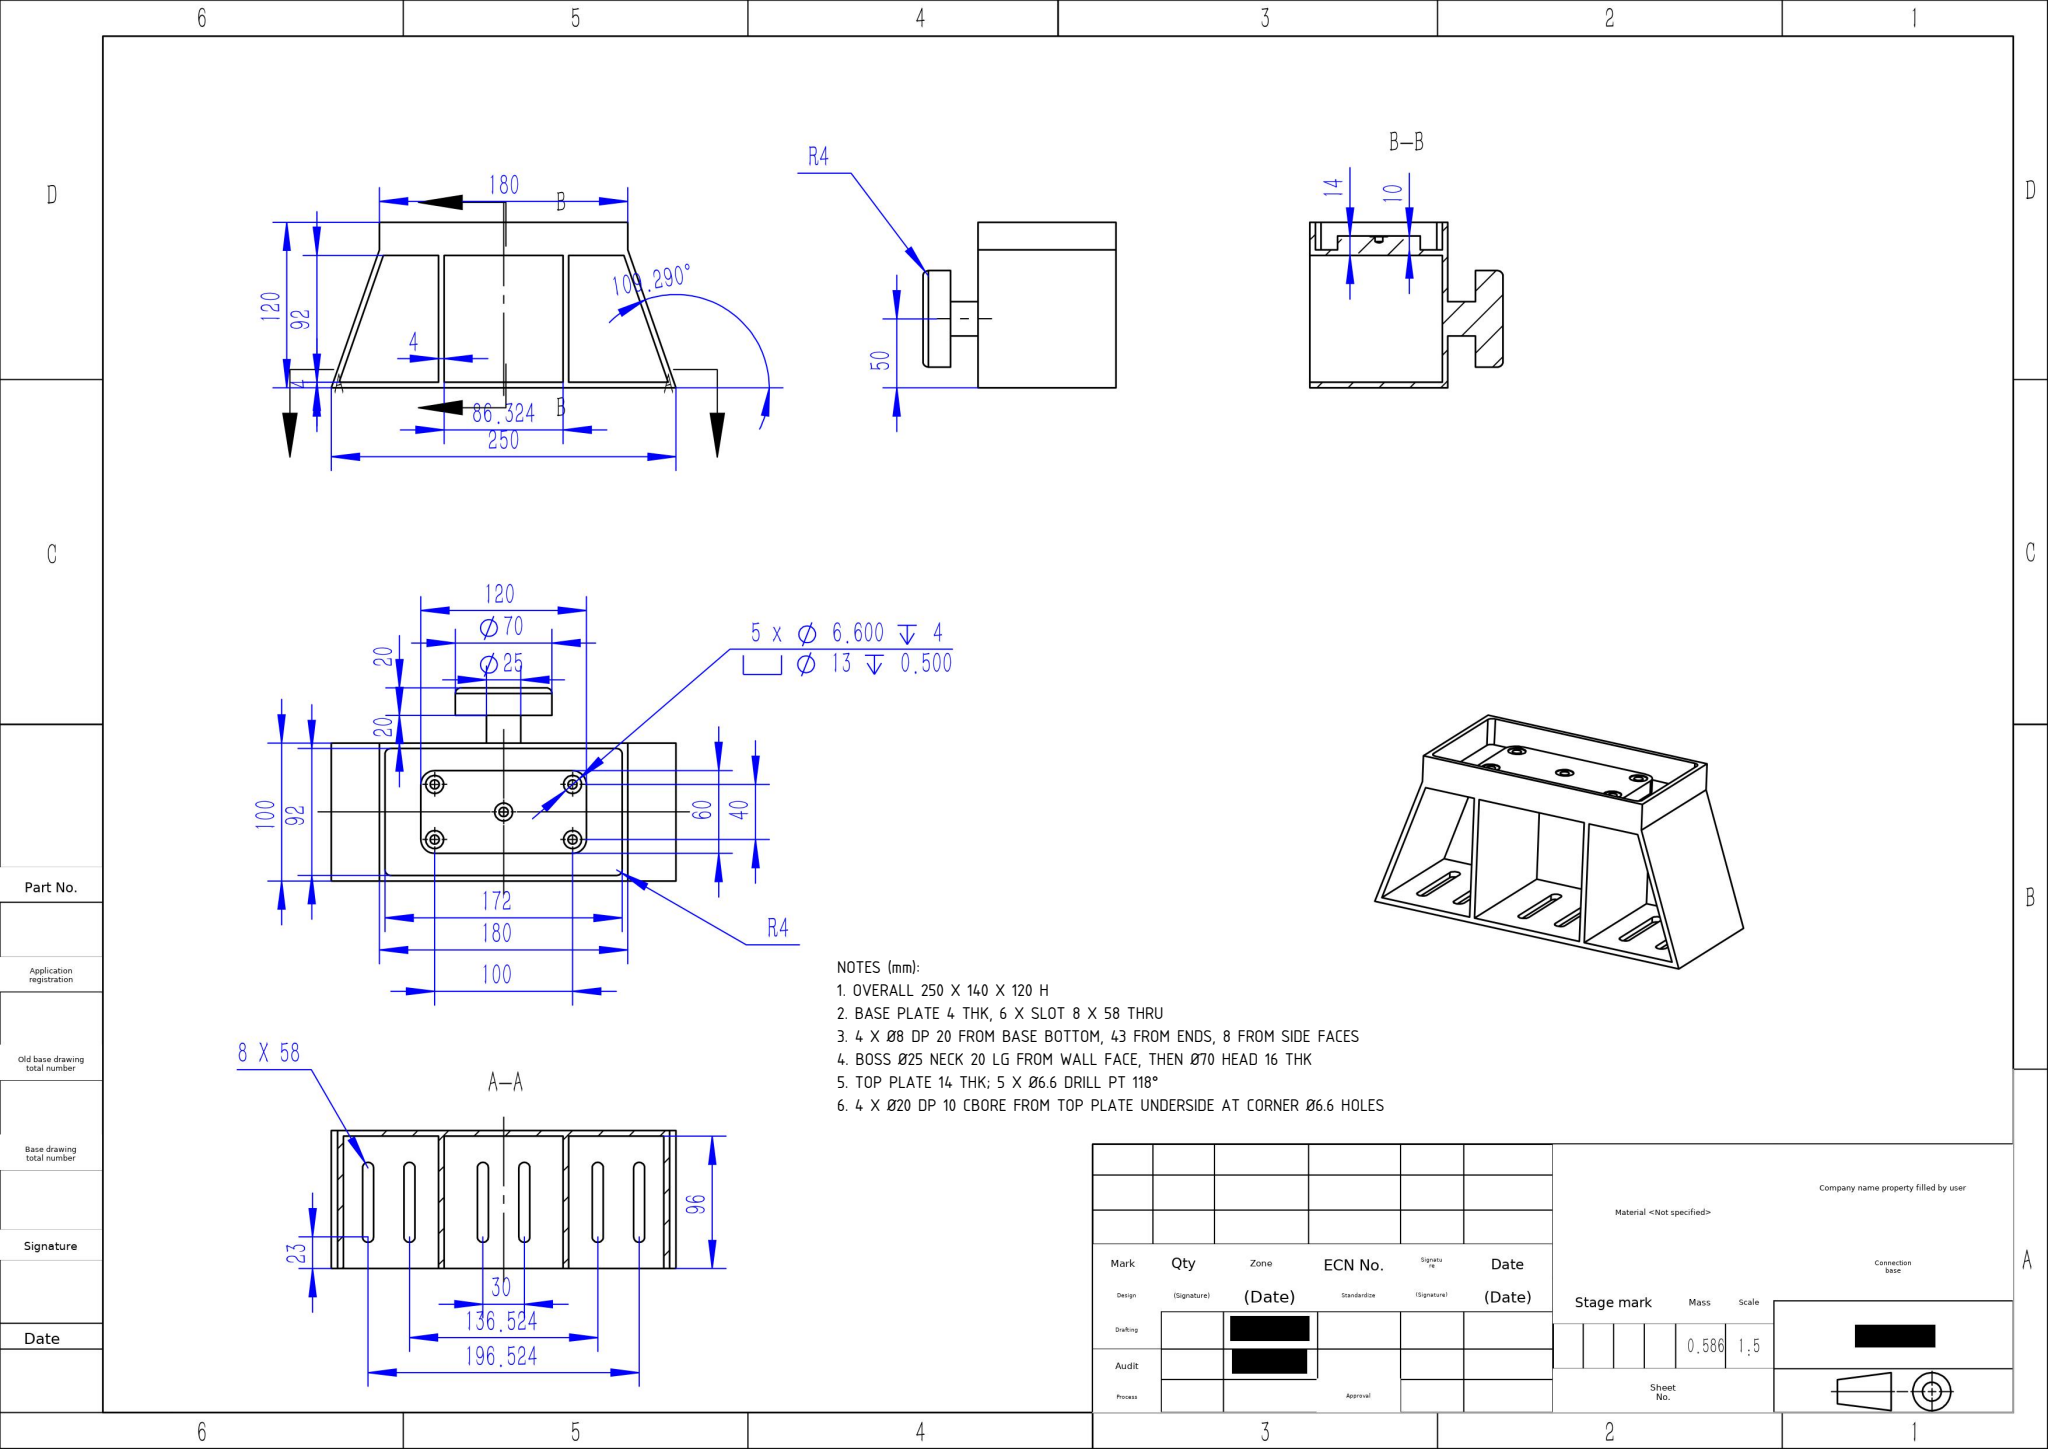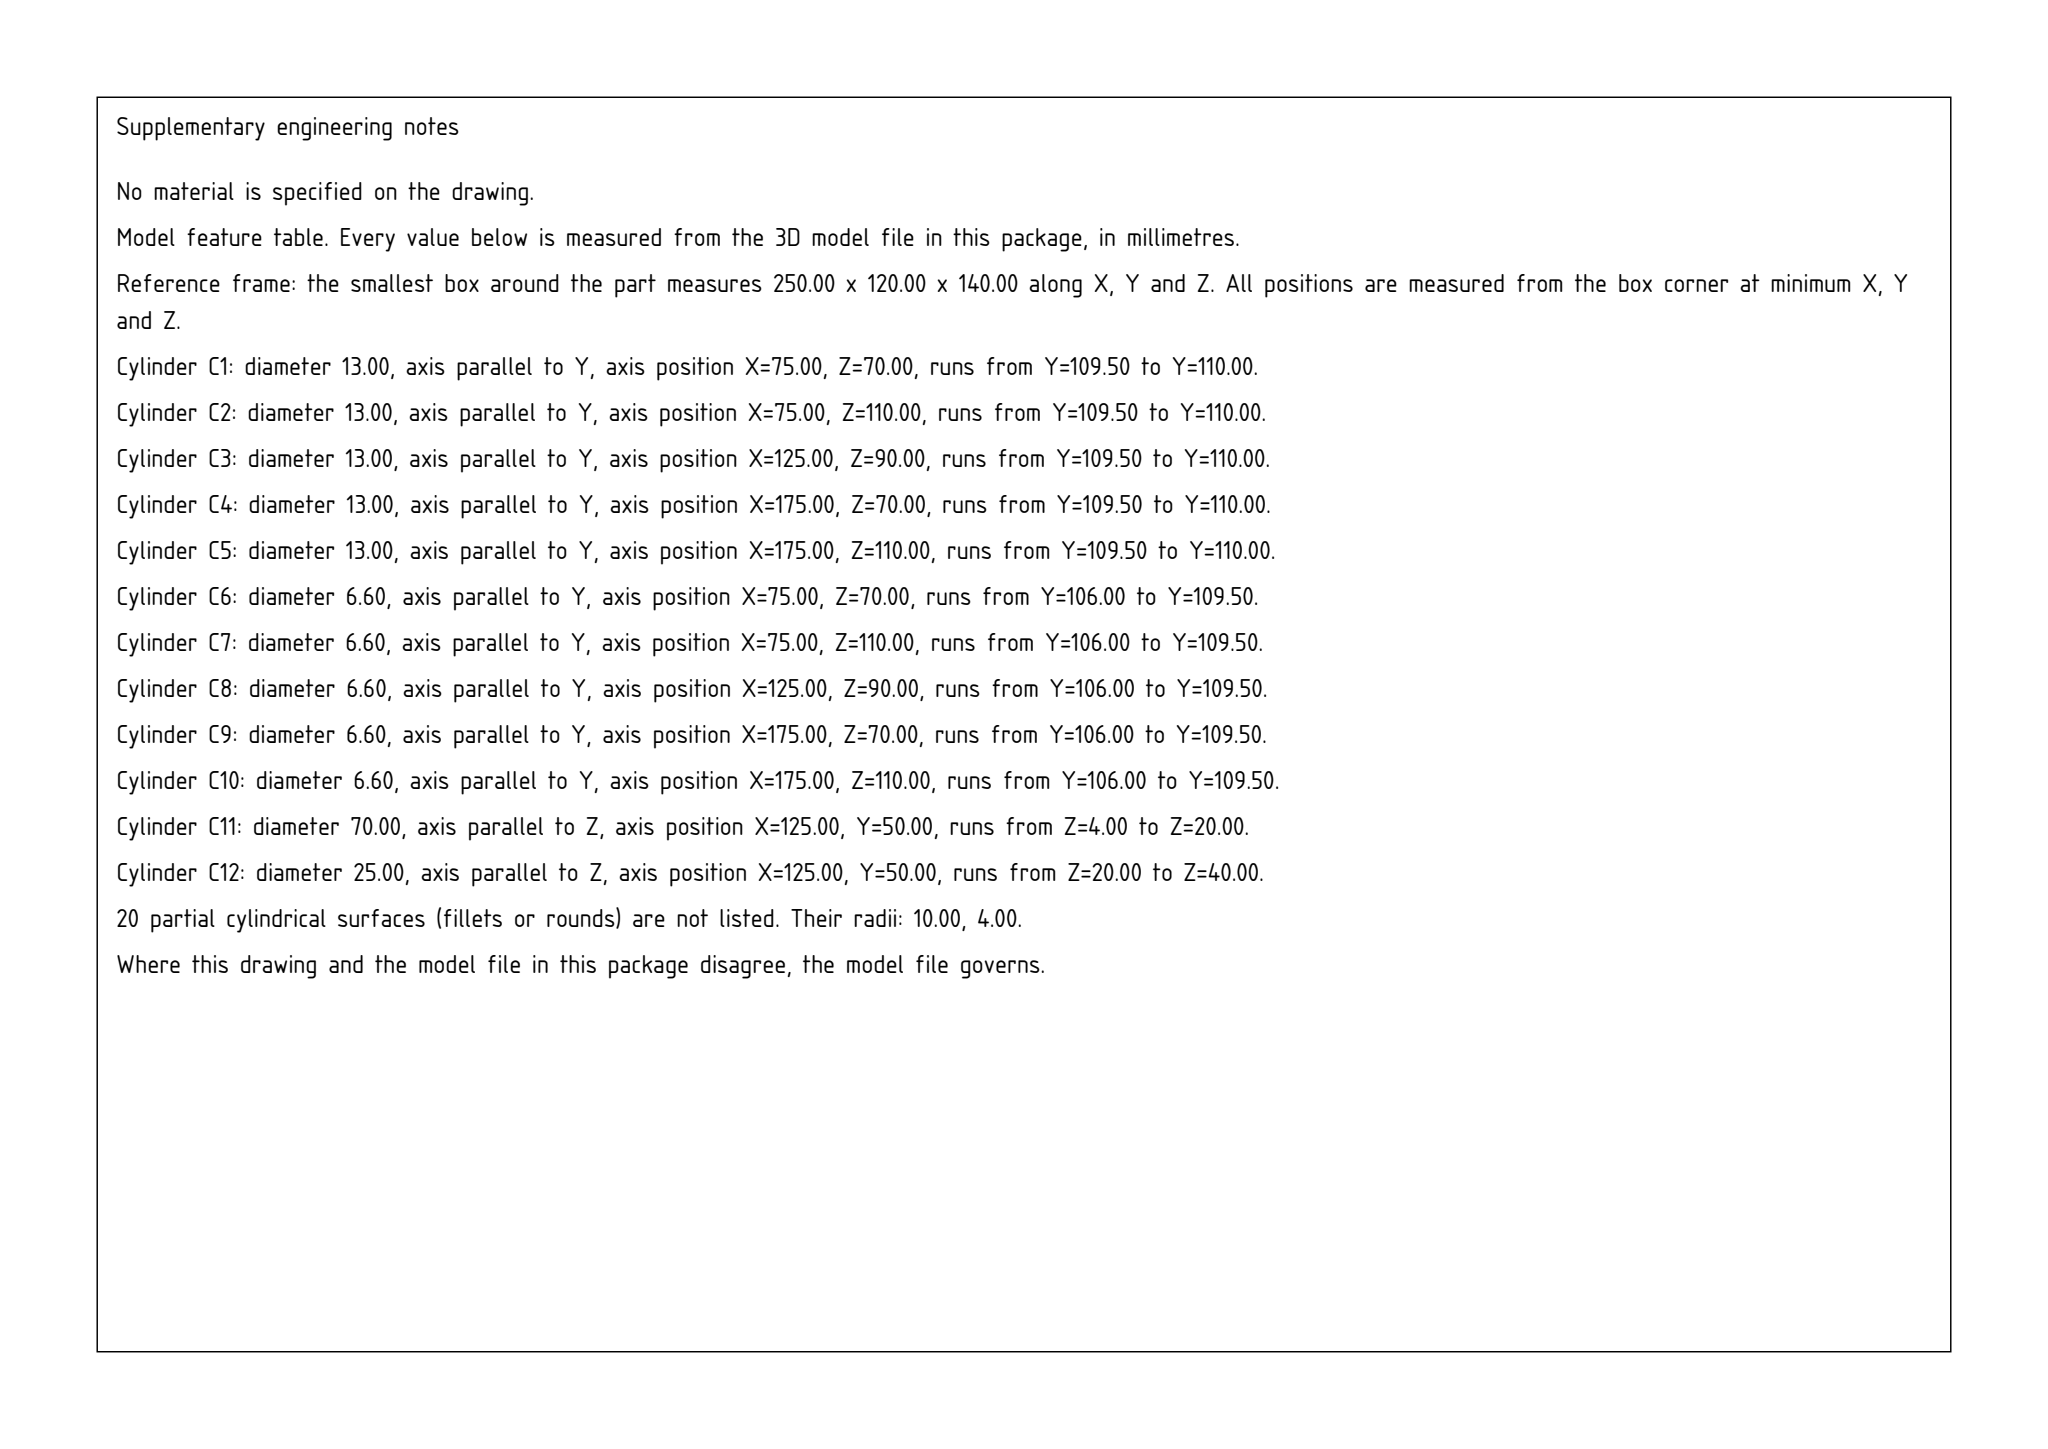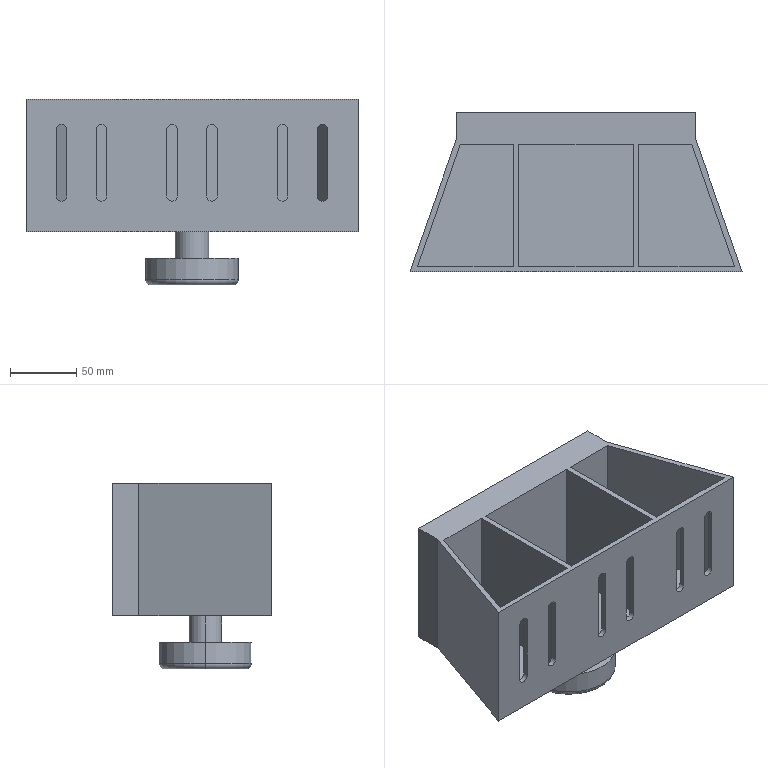Part | SolidWorks | mm | 1 solid | 108 faces | box 250 x 120 x 140 mm | volume 585772 mm3 | plane 52 | cylinder 44 | cone 10 | torus 2 | commonest cylinder face diameters 8 x16 13 x10 6.6 x10 20 x4 70 x2 25 x2
Drawing notes:
OVERALL 250 X 140 X 120 H | from the solid: bbox_xyz 250 x 120 x 140
BASE PLATE 4 THK, 6 X SLOT 8 X 58 THRU | from the solid: Ø8 y-axis cyls L=4 at z=67 & 117 (58 over ends), x=26.74/56.74, 110/140, 193.26/223.26; y planes 0 & 4
4 X Ø8 DP 20 FROM BASE BOTTOM, 43 FROM ENDS, 8 FROM SIDE FACES | from the solid: Ø8 y-axis cyls L=20 at x=43 & 207, z=48 & 132 (outer faces z=40/140), y 0-20
BOSS Ø25 NECK 20 LG FROM WALL FACE, THEN Ø70 HEAD 16 THK | from the solid: Ø25 z-axis cyl L=20 and Ø70 z-axis cyl L=16 at x=125, y=50; wall face z=40, step z=20
TOP PLATE 14 THK; 5 X Ø6.6 DRILL PT 118° | from the solid: y planes 96 (underside) & 110 (top) = 14 thk; cone 118° on Ø6.6 holes
4 X Ø20 DP 10 CBORE FROM TOP PLATE UNDERSIDE AT CORNER Ø6.6 HOLES | from the solid: Ø20 y-axis cyls L=10 at (x,z)=(75,70),(75,110),(175,70),(175,110), y 96-106
build123d program:
from build123d import *

# Parameters (mm, degrees)
BOSS_EXTRUDE1_DEPTH                           = 50
SKETCH2_W                                     = 86.324
SKETCH2_H                                     = 92
CUT_EXTRUDE1_DEPTH                            = 96
SKETCH3_W                                     = 180
SKETCH3_H                                     = 100
SKETCH3_W_2                                   = 172
SKETCH3_H_2                                   = 92
BOSS_EXTRUDE2_DEPTH                           = 20
CUT_EXTRUDE2_DEPTH                            = 20
FILLET1_R                                     = 4
BOSS_EXTRUDE3_DEPTH                           = 10
COUNTERBORE_FOR_M6_HEX_HEAD_BOLT1_D           = 6.6
COUNTERBORE_FOR_M6_HEX_HEAD_BOLT1_DEPTH       = 4
COUNTERBORE_FOR_M6_HEX_HEAD_BOLT1_CBORE_D     = 13
COUNTERBORE_FOR_M6_HEX_HEAD_BOLT1_CBORE_DEPTH = 0.5
COUNTERBORE_FOR_M6_HEX_HEAD_BOLT1_TIP         = 1.983
SKETCH9_R                                     = 12.5
BOSS_EXTRUDE4_DEPTH                           = 20
SKETCH10_R                                    = 35
BOSS_EXTRUDE5_DEPTH                           = 20
FILLET2_R                                     = 4


with BuildPart() as part:
    # Sketch1 → Boss-Extrude1 (new, symmetric)
    with BuildSketch(Plane.XY):
        Polygon((125, 0), (-125, 0), (-90, 100), (90, 100), align=None)
    extrude(amount=BOSS_EXTRUDE1_DEPTH, both=True)

    # Sketch2 → Cut-Extrude1 (cut)
    with BuildSketch(Plane.XY.offset(50)):
        Polygon((-47.162, 96), (-47.162, 4), (-119.362, 4), (-87.162, 96), align=None)
        Polygon((47.162, 96), (47.162, 4), (119.362, 4), (87.162, 96), align=None)
        with Locations((0, 50)):
            Rectangle(SKETCH2_W, SKETCH2_H)
    extrude(amount=-CUT_EXTRUDE1_DEPTH, mode=Mode.SUBTRACT)

    # Sketch3 → Boss-Extrude2 (add)
    with BuildSketch(Plane(origin=(0, 100, 0), x_dir=(1, 0, 0), z_dir=(0, 1, 0))):
        Rectangle(SKETCH3_W, SKETCH3_H)
        Rectangle(SKETCH3_W_2, SKETCH3_H_2, mode=Mode.SUBTRACT)
    extrude(amount=BOSS_EXTRUDE2_DEPTH)

    # Sketch4 → Cut-Extrude2 (cut)
    with BuildSketch(Plane(origin=(0, 4, 0), x_dir=(1, 0, 0), z_dir=(0, 1, 0))):
        with BuildLine():
            Line((-94.262, 23), (-94.262, -27))
            ThreePointArc((-94.262, -27), (-98.262, -31), (-102.262, -27))
            Line((-102.262, -27), (-102.262, 23))
            ThreePointArc((-102.262, 23), (-98.262, 27), (-94.262, 23))
        make_face()
        with BuildLine():
            Line((-64.262, 23), (-64.262, -27))
            ThreePointArc((-64.262, -27), (-68.262, -31), (-72.262, -27))
            Line((-72.262, -27), (-72.262, 23))
            ThreePointArc((-72.262, 23), (-68.262, 27), (-64.262, 23))
        make_face()
        with BuildLine():
            Line((-11, 23), (-11, -27))
            ThreePointArc((-11, -27), (-15, -31), (-19, -27))
            Line((-19, -27), (-19, 23))
            ThreePointArc((-19, 23), (-15, 27), (-11, 23))
        make_face()
        with BuildLine():
            Line((19, 23), (19, -27))
            ThreePointArc((19, -27), (15, -31), (11, -27))
            Line((11, -27), (11, 23))
            ThreePointArc((11, 23), (15, 27), (19, 23))
        make_face()
        with BuildLine():
            Line((72.262, 23), (72.262, -27))
            ThreePointArc((72.262, -27), (68.262, -31), (64.262, -27))
            Line((64.262, -27), (64.262, 23))
            ThreePointArc((64.262, 23), (68.262, 27), (72.262, 23))
        make_face()
        with BuildLine():
            Line((102.262, 23), (102.262, -27))
            ThreePointArc((102.262, -27), (98.262, -31), (94.262, -27))
            Line((94.262, -27), (94.262, 23))
            ThreePointArc((94.262, 23), (98.262, 27), (102.262, 23))
        make_face()
    extrude(amount=-CUT_EXTRUDE2_DEPTH, mode=Mode.SUBTRACT)

    # Fillet1
    fillet1_edges = [part.edges().sort_by_distance(p)[0] for p in [
        (86, 110, 46),
        (86, 110, -46),
        (-86, 110, -46),
        (-86, 110, 46),
    ]]
    fillet(fillet1_edges, radius=FILLET1_R)

    # Sketch5 → Boss-Extrude3 (add)
    with BuildSketch(Plane(origin=(0, 100, 0), x_dir=(1, 0, 0), z_dir=(0, 1, 0))):
        with BuildLine():
            Line((-50, -30), (50, -30))
            ThreePointArc((50, -30), (57.071, -27.071), (60, -20))
            Line((60, -20), (60, 20))
            ThreePointArc((60, 20), (57.071, 27.071), (50, 30))
            Line((50, 30), (-50, 30))
            ThreePointArc((-50, 30), (-57.071, 27.071), (-60, 20))
            Line((-60, 20), (-60, -20))
            ThreePointArc((-60, -20), (-57.071, -27.071), (-50, -30))
        make_face()
    extrude(amount=BOSS_EXTRUDE3_DEPTH)

    # Counterbore for M6 Hex Head Bolt1
    with Locations(Plane(origin=(0, 110, 0), x_dir=(1, 0, 0), z_dir=(0, 1, 0))):
        with Locations((-50, 20), (-50, -20), (50, -20), (50, 20), (0, 0)):
            CounterBoreHole(COUNTERBORE_FOR_M6_HEX_HEAD_BOLT1_D / 2, COUNTERBORE_FOR_M6_HEX_HEAD_BOLT1_CBORE_D / 2, COUNTERBORE_FOR_M6_HEX_HEAD_BOLT1_CBORE_DEPTH, depth=COUNTERBORE_FOR_M6_HEX_HEAD_BOLT1_DEPTH)
            with Locations((0, 0, -(COUNTERBORE_FOR_M6_HEX_HEAD_BOLT1_DEPTH + COUNTERBORE_FOR_M6_HEX_HEAD_BOLT1_TIP / 2))):  # 118° drill point
                Cone(0, COUNTERBORE_FOR_M6_HEX_HEAD_BOLT1_D / 2, COUNTERBORE_FOR_M6_HEX_HEAD_BOLT1_TIP, mode=Mode.SUBTRACT)

    # Sketch9 → Boss-Extrude4 (add)
    with BuildSketch(Plane(origin=(0, 0, -50), x_dir=(-1, 0, 0), z_dir=(0, 0, -1))):
        with Locations((0, 50)):
            Circle(SKETCH9_R)
    extrude(amount=BOSS_EXTRUDE4_DEPTH)

    # Sketch10 → Boss-Extrude5 (add)
    with BuildSketch(Plane(origin=(0, 0, -70), x_dir=(-1, 0, 0), z_dir=(0, 0, -1))):
        with Locations((0, 50)):
            Circle(SKETCH10_R)
    extrude(amount=BOSS_EXTRUDE5_DEPTH)

    # Fillet2
    fillet2_edges = [part.edges().sort_by_distance(p)[0] for p in [
        (35, 50, -90),
    ]]
    fillet(fillet2_edges, radius=FILLET2_R)


solid = part.part